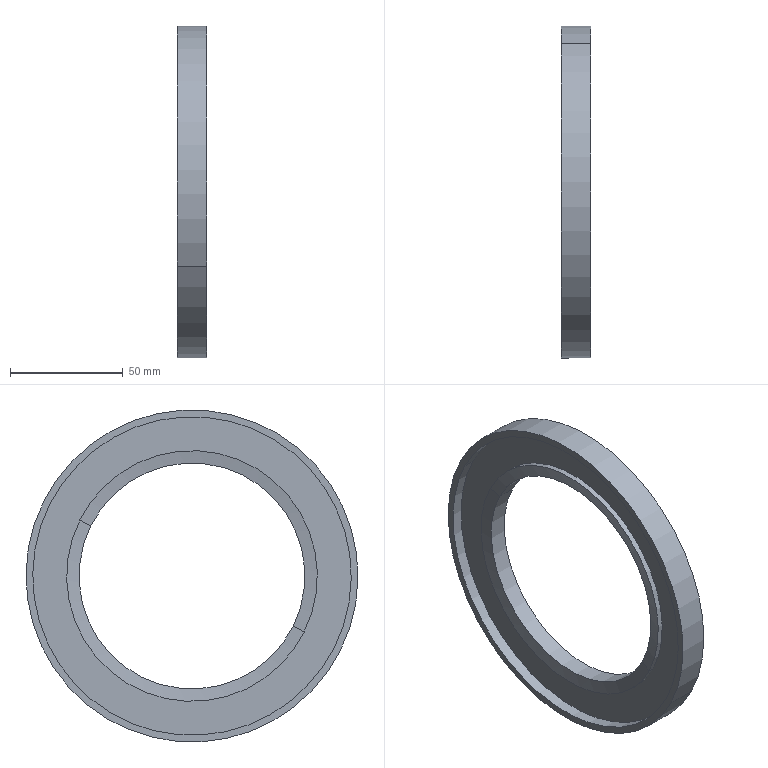Component | SolidWorks | SpringSeat-1 | 1 solid | 16 faces | box 13 x 147 x 147 mm | volume 74131 mm3 | cylinder 10 | plane 4 | cone 2 | commonest cylinder face diameters 141 x2 111 x2 100 x2 134 x2 147 x2
build123d program:
from build123d import *


with BuildPart() as part:
    # Sketch1 → Revolve1 (revolve)
    with BuildSketch(Plane.XY, mode=Mode.PRIVATE) as revolve1_sk:
        Polygon((0, 73.5), (13, 73.5), (13, 67), (11.5, 67), (11.5, 50), (3.371, 50), (2.5, 55.5), (5, 55.5), (5, 70.5), (0, 70.5), align=None)
    revolve(revolve1_sk.sketch.rotate(Axis((0, 0, 0), (1, 0, 0)), 90), axis=Axis((0, 0, 0), (1, 0, 0)))


solid = part.part

# Placed as in the assembly
solid = solid.moved(Location((-149.5, 0, 0), (0, 0, 0)))
STEP:
#1=COLOUR_RGB('',0.7922,0.8196,0.9333);
#2=FILL_AREA_STYLE_COLOUR('',#1);
#3=FILL_AREA_STYLE('',(#2));
#4=SURFACE_STYLE_FILL_AREA(#3);
#5=SURFACE_SIDE_STYLE('',(#4));
#6=SURFACE_STYLE_USAGE(.BOTH.,#5);
#7=PRESENTATION_STYLE_ASSIGNMENT((#6));
#8=CARTESIAN_POINT('',(-5.689,-2.483,-1.24));
#9=VERTEX_POINT('',#8);
#10=CARTESIAN_POINT('',(-5.689,2.483,1.24));
#11=VERTEX_POINT('',#10);
#12=CARTESIAN_POINT('',(-5.689,-0.,0.));
#13=DIRECTION('',(-1.,-0.,0.));
#14=DIRECTION('',(-0.,0.8946,0.4468));
#15=AXIS2_PLACEMENT_3D('',#12,#13,#14);
#16=CIRCLE('',#15,2.776);
#17=EDGE_CURVE('',#9,#11,#16,.T.);
#18=ORIENTED_EDGE('',*,*,#17,.F.);
#19=CARTESIAN_POINT('',(-5.886,-2.483,-1.24));
#20=VERTEX_POINT('',#19);
#21=CARTESIAN_POINT('',(-5.886,-2.483,-1.24));
#22=DIRECTION('',(-1.,-0.,0.));
#23=VECTOR('',#22,39.37);
#24=LINE('',#21,#23);
#25=EDGE_CURVE('',#9,#20,#24,.T.);
#26=ORIENTED_EDGE('',*,*,#25,.T.);
#27=CARTESIAN_POINT('',(-5.886,2.483,1.24));
#28=VERTEX_POINT('',#27);
#29=CARTESIAN_POINT('',(-5.886,-0.,0.));
#30=DIRECTION('',(-1.,-0.,0.));
#31=DIRECTION('',(-0.,0.8946,0.4468));
#32=AXIS2_PLACEMENT_3D('',#29,#30,#31);
#33=CIRCLE('',#32,2.776);
#34=EDGE_CURVE('',#20,#28,#33,.T.);
#35=ORIENTED_EDGE('',*,*,#34,.T.);
#36=CARTESIAN_POINT('',(-5.886,2.483,1.24));
#37=DIRECTION('',(-1.,-0.,0.));
#38=VECTOR('',#37,39.37);
#39=LINE('',#36,#38);
#40=EDGE_CURVE('',#11,#28,#39,.T.);
#41=ORIENTED_EDGE('',*,*,#40,.F.);
#42=EDGE_LOOP('',(#18,#26,#35,#41));
#43=FACE_OUTER_BOUND('',#42,.T.);
#44=CARTESIAN_POINT('',(-5.886,-0.,0.));
#45=DIRECTION('',(-1.,-0.,0.));
#46=DIRECTION('',(-0.,0.8946,0.4468));
#47=AXIS2_PLACEMENT_3D('',#44,#45,#46);
#48=CYLINDRICAL_SURFACE('',#47,2.776);
#49=ADVANCED_FACE('',(#43),#48,.F.);
#50=CARTESIAN_POINT('',(-5.689,1.955,0.9764));
#51=VERTEX_POINT('',#50);
#52=CARTESIAN_POINT('',(-5.689,-1.955,-0.9764));
#53=VERTEX_POINT('',#52);
#54=CARTESIAN_POINT('',(-5.689,-0.,0.));
#55=DIRECTION('',(-1.,-0.,0.));
#56=DIRECTION('',(-0.,0.8946,0.4468));
#57=AXIS2_PLACEMENT_3D('',#54,#55,#56);
#58=CIRCLE('',#57,2.185);
#59=EDGE_CURVE('',#51,#53,#58,.T.);
#60=ORIENTED_EDGE('',*,*,#59,.T.);
#61=CARTESIAN_POINT('',(-5.787,-1.955,-0.9764));
#62=VERTEX_POINT('',#61);
#63=CARTESIAN_POINT('',(-5.886,-1.955,-0.9764));
#64=DIRECTION('',(-1.,-0.,0.));
#65=VECTOR('',#64,39.37);
#66=LINE('',#63,#65);
#67=EDGE_CURVE('',#53,#62,#66,.T.);
#68=ORIENTED_EDGE('',*,*,#67,.T.);
#69=CARTESIAN_POINT('',(-5.787,1.955,0.9764));
#70=VERTEX_POINT('',#69);
#71=CARTESIAN_POINT('',(-5.787,-0.,0.));
#72=DIRECTION('',(-1.,-0.,0.));
#73=DIRECTION('',(-0.,0.8946,0.4468));
#74=AXIS2_PLACEMENT_3D('',#71,#72,#73);
#75=CIRCLE('',#74,2.185);
#76=EDGE_CURVE('',#70,#62,#75,.T.);
#77=ORIENTED_EDGE('',*,*,#76,.F.);
#78=CARTESIAN_POINT('',(-5.886,1.955,0.9764));
#79=DIRECTION('',(-1.,-0.,0.));
#80=VECTOR('',#79,39.37);
#81=LINE('',#78,#80);
#82=EDGE_CURVE('',#51,#70,#81,.T.);
#83=ORIENTED_EDGE('',*,*,#82,.F.);
#84=EDGE_LOOP('',(#60,#68,#77,#83));
#85=FACE_OUTER_BOUND('',#84,.T.);
#86=CARTESIAN_POINT('',(-5.886,-0.,0.));
#87=DIRECTION('',(-1.,-0.,0.));
#88=DIRECTION('',(-0.,0.8946,0.4468));
#89=AXIS2_PLACEMENT_3D('',#86,#87,#88);
#90=CYLINDRICAL_SURFACE('',#89,2.185);
#91=ADVANCED_FACE('',(#85),#90,.T.);
#92=CARTESIAN_POINT('',(-5.753,-1.761,-0.8796));
#93=VERTEX_POINT('',#92);
#94=CARTESIAN_POINT('',(-5.753,1.761,0.8796));
#95=VERTEX_POINT('',#94);
#96=CARTESIAN_POINT('',(-5.753,-0.,0.));
#97=DIRECTION('',(-1.,-0.,0.));
#98=DIRECTION('',(-0.,0.8946,0.4468));
#99=AXIS2_PLACEMENT_3D('',#96,#97,#98);
#100=CIRCLE('',#99,1.969);
#101=EDGE_CURVE('',#93,#95,#100,.T.);
#102=ORIENTED_EDGE('',*,*,#101,.F.);
#103=CARTESIAN_POINT('',(-5.787,-1.955,-0.9764));
#104=DIRECTION('',(-0.1564,-0.8836,-0.4413));
#105=VECTOR('',#104,39.37);
#106=LINE('',#103,#105);
#107=EDGE_CURVE('',#93,#62,#106,.T.);
#108=ORIENTED_EDGE('',*,*,#107,.T.);
#109=CARTESIAN_POINT('',(-5.787,-0.,0.));
#110=DIRECTION('',(-1.,-0.,0.));
#111=DIRECTION('',(-0.,0.8946,0.4468));
#112=AXIS2_PLACEMENT_3D('',#109,#110,#111);
#113=CIRCLE('',#112,2.185);
#114=EDGE_CURVE('',#62,#70,#113,.T.);
#115=ORIENTED_EDGE('',*,*,#114,.T.);
#116=CARTESIAN_POINT('',(-5.787,1.955,0.9764));
#117=DIRECTION('',(-0.1564,0.8836,0.4413));
#118=VECTOR('',#117,39.37);
#119=LINE('',#116,#118);
#120=EDGE_CURVE('',#95,#70,#119,.T.);
#121=ORIENTED_EDGE('',*,*,#120,.F.);
#122=EDGE_LOOP('',(#102,#108,#115,#121));
#123=FACE_OUTER_BOUND('',#122,.T.);
#124=CARTESIAN_POINT('',(-5.787,-0.,0.));
#125=DIRECTION('',(-1.,-0.,0.));
#126=DIRECTION('',(-0.,0.8946,0.4468));
#127=AXIS2_PLACEMENT_3D('',#124,#125,#126);
#128=CONICAL_SURFACE('',#127,2.185,1.414);
#129=ADVANCED_FACE('',(#123),#128,.F.);
#130=CARTESIAN_POINT('',(-5.433,-1.761,-0.8796));
#131=VERTEX_POINT('',#130);
#132=CARTESIAN_POINT('',(-5.433,1.761,0.8796));
#133=VERTEX_POINT('',#132);
#134=CARTESIAN_POINT('',(-5.433,-0.,0.));
#135=DIRECTION('',(-1.,-0.,0.));
#136=DIRECTION('',(-0.,0.8946,0.4468));
#137=AXIS2_PLACEMENT_3D('',#134,#135,#136);
#138=CIRCLE('',#137,1.969);
#139=EDGE_CURVE('',#131,#133,#138,.T.);
#140=ORIENTED_EDGE('',*,*,#139,.F.);
#141=CARTESIAN_POINT('',(-5.886,-1.761,-0.8796));
#142=DIRECTION('',(-1.,-0.,0.));
#143=VECTOR('',#142,39.37);
#144=LINE('',#141,#143);
#145=EDGE_CURVE('',#131,#93,#144,.T.);
#146=ORIENTED_EDGE('',*,*,#145,.T.);
#147=ORIENTED_EDGE('',*,*,#101,.T.);
#148=CARTESIAN_POINT('',(-5.886,1.761,0.8796));
#149=DIRECTION('',(-1.,-0.,0.));
#150=VECTOR('',#149,39.37);
#151=LINE('',#148,#150);
#152=EDGE_CURVE('',#133,#95,#151,.T.);
#153=ORIENTED_EDGE('',*,*,#152,.F.);
#154=EDGE_LOOP('',(#140,#146,#147,#153));
#155=FACE_OUTER_BOUND('',#154,.T.);
#156=CARTESIAN_POINT('',(-5.886,-0.,0.));
#157=DIRECTION('',(-1.,-0.,0.));
#158=DIRECTION('',(-0.,0.8946,0.4468));
#159=AXIS2_PLACEMENT_3D('',#156,#157,#158);
#160=CYLINDRICAL_SURFACE('',#159,1.969);
#161=ADVANCED_FACE('',(#155),#160,.F.);
#162=CARTESIAN_POINT('',(-5.374,-2.36,-1.179));
#163=VERTEX_POINT('',#162);
#164=CARTESIAN_POINT('',(-5.374,2.36,1.179));
#165=VERTEX_POINT('',#164);
#166=CARTESIAN_POINT('',(-5.374,-0.,0.));
#167=DIRECTION('',(-1.,-0.,0.));
#168=DIRECTION('',(-0.,0.8946,0.4468));
#169=AXIS2_PLACEMENT_3D('',#166,#167,#168);
#170=CIRCLE('',#169,2.638);
#171=EDGE_CURVE('',#163,#165,#170,.T.);
#172=ORIENTED_EDGE('',*,*,#171,.F.);
#173=CARTESIAN_POINT('',(-5.433,-2.36,-1.179));
#174=VERTEX_POINT('',#173);
#175=CARTESIAN_POINT('',(-5.886,-2.36,-1.179));
#176=DIRECTION('',(-1.,-0.,0.));
#177=VECTOR('',#176,39.37);
#178=LINE('',#175,#177);
#179=EDGE_CURVE('',#163,#174,#178,.T.);
#180=ORIENTED_EDGE('',*,*,#179,.T.);
#181=CARTESIAN_POINT('',(-5.433,2.36,1.179));
#182=VERTEX_POINT('',#181);
#183=CARTESIAN_POINT('',(-5.433,-0.,0.));
#184=DIRECTION('',(-1.,-0.,0.));
#185=DIRECTION('',(-0.,0.8946,0.4468));
#186=AXIS2_PLACEMENT_3D('',#183,#184,#185);
#187=CIRCLE('',#186,2.638);
#188=EDGE_CURVE('',#174,#182,#187,.T.);
#189=ORIENTED_EDGE('',*,*,#188,.T.);
#190=CARTESIAN_POINT('',(-5.886,2.36,1.179));
#191=DIRECTION('',(-1.,-0.,0.));
#192=VECTOR('',#191,39.37);
#193=LINE('',#190,#192);
#194=EDGE_CURVE('',#165,#182,#193,.T.);
#195=ORIENTED_EDGE('',*,*,#194,.F.);
#196=EDGE_LOOP('',(#172,#180,#189,#195));
#197=FACE_OUTER_BOUND('',#196,.T.);
#198=CARTESIAN_POINT('',(-5.886,-0.,0.));
#199=DIRECTION('',(-1.,-0.,0.));
#200=DIRECTION('',(-0.,0.8946,0.4468));
#201=AXIS2_PLACEMENT_3D('',#198,#199,#200);
#202=CYLINDRICAL_SURFACE('',#201,2.638);
#203=ADVANCED_FACE('',(#197),#202,.F.);
#204=CARTESIAN_POINT('',(-5.374,2.589,1.293));
#205=VERTEX_POINT('',#204);
#206=CARTESIAN_POINT('',(-5.374,-2.589,-1.293));
#207=VERTEX_POINT('',#206);
#208=CARTESIAN_POINT('',(-5.374,-0.,0.));
#209=DIRECTION('',(-1.,-0.,0.));
#210=DIRECTION('',(-0.,0.8946,0.4468));
#211=AXIS2_PLACEMENT_3D('',#208,#209,#210);
#212=CIRCLE('',#211,2.894);
#213=EDGE_CURVE('',#205,#207,#212,.T.);
#214=ORIENTED_EDGE('',*,*,#213,.T.);
#215=CARTESIAN_POINT('',(-5.886,-2.589,-1.293));
#216=VERTEX_POINT('',#215);
#217=CARTESIAN_POINT('',(-5.886,-2.589,-1.293));
#218=DIRECTION('',(-1.,-0.,0.));
#219=VECTOR('',#218,39.37);
#220=LINE('',#217,#219);
#221=EDGE_CURVE('',#207,#216,#220,.T.);
#222=ORIENTED_EDGE('',*,*,#221,.T.);
#223=CARTESIAN_POINT('',(-5.886,2.589,1.293));
#224=VERTEX_POINT('',#223);
#225=CARTESIAN_POINT('',(-5.886,-0.,0.));
#226=DIRECTION('',(-1.,-0.,0.));
#227=DIRECTION('',(-0.,0.8946,0.4468));
#228=AXIS2_PLACEMENT_3D('',#225,#226,#227);
#229=CIRCLE('',#228,2.894);
#230=EDGE_CURVE('',#224,#216,#229,.T.);
#231=ORIENTED_EDGE('',*,*,#230,.F.);
#232=CARTESIAN_POINT('',(-5.886,2.589,1.293));
#233=DIRECTION('',(-1.,-0.,0.));
#234=VECTOR('',#233,39.37);
#235=LINE('',#232,#234);
#236=EDGE_CURVE('',#205,#224,#235,.T.);
#237=ORIENTED_EDGE('',*,*,#236,.F.);
#238=EDGE_LOOP('',(#214,#222,#231,#237));
#239=FACE_OUTER_BOUND('',#238,.T.);
#240=CARTESIAN_POINT('',(-5.886,-0.,0.));
#241=DIRECTION('',(-1.,-0.,0.));
#242=DIRECTION('',(-0.,0.8946,0.4468));
#243=AXIS2_PLACEMENT_3D('',#240,#241,#242);
#244=CYLINDRICAL_SURFACE('',#243,2.894);
#245=ADVANCED_FACE('',(#239),#244,.T.);
#246=CARTESIAN_POINT('',(-5.886,-0.,0.));
#247=DIRECTION('',(-1.,-0.,0.));
#248=DIRECTION('',(-0.,0.8946,0.4468));
#249=AXIS2_PLACEMENT_3D('',#246,#247,#248);
#250=CIRCLE('',#249,2.776);
#251=EDGE_CURVE('',#28,#20,#250,.T.);
#252=ORIENTED_EDGE('',*,*,#251,.F.);
#253=ORIENTED_EDGE('',*,*,#34,.F.);
#254=EDGE_LOOP('',(#252,#253));
#255=FACE_BOUND('',#254,.T.);
#256=ORIENTED_EDGE('',*,*,#230,.T.);
#257=CARTESIAN_POINT('',(-5.886,-0.,0.));
#258=DIRECTION('',(-1.,-0.,0.));
#259=DIRECTION('',(-0.,0.8946,0.4468));
#260=AXIS2_PLACEMENT_3D('',#257,#258,#259);
#261=CIRCLE('',#260,2.894);
#262=EDGE_CURVE('',#216,#224,#261,.T.);
#263=ORIENTED_EDGE('',*,*,#262,.T.);
#264=EDGE_LOOP('',(#256,#263));
#265=FACE_OUTER_BOUND('',#264,.T.);
#266=CARTESIAN_POINT('',(-5.886,1.24,-2.483));
#267=DIRECTION('',(1.,0.,-0.));
#268=DIRECTION('',(0.,-0.8946,-0.4468));
#269=AXIS2_PLACEMENT_3D('',#266,#267,#268);
#270=PLANE('',#269);
#271=ADVANCED_FACE('',(#255,#265),#270,.F.);
#272=ORIENTED_EDGE('',*,*,#221,.F.);
#273=CARTESIAN_POINT('',(-5.374,-0.,0.));
#274=DIRECTION('',(-1.,-0.,0.));
#275=DIRECTION('',(-0.,0.8946,0.4468));
#276=AXIS2_PLACEMENT_3D('',#273,#274,#275);
#277=CIRCLE('',#276,2.894);
#278=EDGE_CURVE('',#207,#205,#277,.T.);
#279=ORIENTED_EDGE('',*,*,#278,.T.);
#280=ORIENTED_EDGE('',*,*,#236,.T.);
#281=ORIENTED_EDGE('',*,*,#262,.F.);
#282=EDGE_LOOP('',(#272,#279,#280,#281));
#283=FACE_OUTER_BOUND('',#282,.T.);
#284=CARTESIAN_POINT('',(-5.886,-0.,0.));
#285=DIRECTION('',(-1.,-0.,0.));
#286=DIRECTION('',(-0.,0.8946,0.4468));
#287=AXIS2_PLACEMENT_3D('',#284,#285,#286);
#288=CYLINDRICAL_SURFACE('',#287,2.894);
#289=ADVANCED_FACE('',(#283),#288,.T.);
#290=ORIENTED_EDGE('',*,*,#213,.F.);
#291=ORIENTED_EDGE('',*,*,#278,.F.);
#292=EDGE_LOOP('',(#290,#291));
#293=FACE_OUTER_BOUND('',#292,.T.);
#294=CARTESIAN_POINT('',(-5.374,-0.,0.));
#295=DIRECTION('',(-1.,-0.,0.));
#296=DIRECTION('',(-0.,0.8946,0.4468));
#297=AXIS2_PLACEMENT_3D('',#294,#295,#296);
#298=CIRCLE('',#297,2.638);
#299=EDGE_CURVE('',#165,#163,#298,.T.);
#300=ORIENTED_EDGE('',*,*,#299,.T.);
#301=ORIENTED_EDGE('',*,*,#171,.T.);
#302=EDGE_LOOP('',(#300,#301));
#303=FACE_BOUND('',#302,.T.);
#304=CARTESIAN_POINT('',(-5.374,1.293,-2.589));
#305=DIRECTION('',(-1.,-0.,0.));
#306=DIRECTION('',(-0.,0.8946,0.4468));
#307=AXIS2_PLACEMENT_3D('',#304,#305,#306);
#308=PLANE('',#307);
#309=ADVANCED_FACE('',(#293,#303),#308,.F.);
#310=ORIENTED_EDGE('',*,*,#179,.F.);
#311=ORIENTED_EDGE('',*,*,#299,.F.);
#312=ORIENTED_EDGE('',*,*,#194,.T.);
#313=CARTESIAN_POINT('',(-5.433,-0.,0.));
#314=DIRECTION('',(-1.,-0.,0.));
#315=DIRECTION('',(-0.,0.8946,0.4468));
#316=AXIS2_PLACEMENT_3D('',#313,#314,#315);
#317=CIRCLE('',#316,2.638);
#318=EDGE_CURVE('',#182,#174,#317,.T.);
#319=ORIENTED_EDGE('',*,*,#318,.T.);
#320=EDGE_LOOP('',(#310,#311,#312,#319));
#321=FACE_OUTER_BOUND('',#320,.T.);
#322=CARTESIAN_POINT('',(-5.886,-0.,0.));
#323=DIRECTION('',(-1.,-0.,0.));
#324=DIRECTION('',(-0.,0.8946,0.4468));
#325=AXIS2_PLACEMENT_3D('',#322,#323,#324);
#326=CYLINDRICAL_SURFACE('',#325,2.638);
#327=ADVANCED_FACE('',(#321),#326,.F.);
#328=ORIENTED_EDGE('',*,*,#318,.F.);
#329=ORIENTED_EDGE('',*,*,#188,.F.);
#330=EDGE_LOOP('',(#328,#329));
#331=FACE_OUTER_BOUND('',#330,.T.);
#332=CARTESIAN_POINT('',(-5.433,-0.,0.));
#333=DIRECTION('',(-1.,-0.,0.));
#334=DIRECTION('',(-0.,0.8946,0.4468));
#335=AXIS2_PLACEMENT_3D('',#332,#333,#334);
#336=CIRCLE('',#335,1.969);
#337=EDGE_CURVE('',#133,#131,#336,.T.);
#338=ORIENTED_EDGE('',*,*,#337,.T.);
#339=ORIENTED_EDGE('',*,*,#139,.T.);
#340=EDGE_LOOP('',(#338,#339));
#341=FACE_BOUND('',#340,.T.);
#342=CARTESIAN_POINT('',(-5.433,1.179,-2.36));
#343=DIRECTION('',(-1.,-0.,0.));
#344=DIRECTION('',(-0.,0.8946,0.4468));
#345=AXIS2_PLACEMENT_3D('',#342,#343,#344);
#346=PLANE('',#345);
#347=ADVANCED_FACE('',(#331,#341),#346,.F.);
#348=ORIENTED_EDGE('',*,*,#145,.F.);
#349=ORIENTED_EDGE('',*,*,#337,.F.);
#350=ORIENTED_EDGE('',*,*,#152,.T.);
#351=CARTESIAN_POINT('',(-5.753,-0.,0.));
#352=DIRECTION('',(-1.,-0.,0.));
#353=DIRECTION('',(-0.,0.8946,0.4468));
#354=AXIS2_PLACEMENT_3D('',#351,#352,#353);
#355=CIRCLE('',#354,1.969);
#356=EDGE_CURVE('',#95,#93,#355,.T.);
#357=ORIENTED_EDGE('',*,*,#356,.T.);
#358=EDGE_LOOP('',(#348,#349,#350,#357));
#359=FACE_OUTER_BOUND('',#358,.T.);
#360=CARTESIAN_POINT('',(-5.886,-0.,0.));
#361=DIRECTION('',(-1.,-0.,0.));
#362=DIRECTION('',(-0.,0.8946,0.4468));
#363=AXIS2_PLACEMENT_3D('',#360,#361,#362);
#364=CYLINDRICAL_SURFACE('',#363,1.969);
#365=ADVANCED_FACE('',(#359),#364,.F.);
#366=ORIENTED_EDGE('',*,*,#107,.F.);
#367=ORIENTED_EDGE('',*,*,#356,.F.);
#368=ORIENTED_EDGE('',*,*,#120,.T.);
#369=ORIENTED_EDGE('',*,*,#76,.T.);
#370=EDGE_LOOP('',(#366,#367,#368,#369));
#371=FACE_OUTER_BOUND('',#370,.T.);
#372=CARTESIAN_POINT('',(-5.787,-0.,0.));
#373=DIRECTION('',(-1.,-0.,0.));
#374=DIRECTION('',(-0.,0.8946,0.4468));
#375=AXIS2_PLACEMENT_3D('',#372,#373,#374);
#376=CONICAL_SURFACE('',#375,2.185,1.414);
#377=ADVANCED_FACE('',(#371),#376,.F.);
#378=ORIENTED_EDGE('',*,*,#67,.F.);
#379=CARTESIAN_POINT('',(-5.689,-0.,0.));
#380=DIRECTION('',(-1.,-0.,0.));
#381=DIRECTION('',(-0.,0.8946,0.4468));
#382=AXIS2_PLACEMENT_3D('',#379,#380,#381);
#383=CIRCLE('',#382,2.185);
#384=EDGE_CURVE('',#53,#51,#383,.T.);
#385=ORIENTED_EDGE('',*,*,#384,.T.);
#386=ORIENTED_EDGE('',*,*,#82,.T.);
#387=ORIENTED_EDGE('',*,*,#114,.F.);
#388=EDGE_LOOP('',(#378,#385,#386,#387));
#389=FACE_OUTER_BOUND('',#388,.T.);
#390=CARTESIAN_POINT('',(-5.886,-0.,0.));
#391=DIRECTION('',(-1.,-0.,0.));
#392=DIRECTION('',(-0.,0.8946,0.4468));
#393=AXIS2_PLACEMENT_3D('',#390,#391,#392);
#394=CYLINDRICAL_SURFACE('',#393,2.185);
#395=ADVANCED_FACE('',(#389),#394,.T.);
#396=ORIENTED_EDGE('',*,*,#59,.F.);
#397=ORIENTED_EDGE('',*,*,#384,.F.);
#398=EDGE_LOOP('',(#396,#397));
#399=FACE_BOUND('',#398,.T.);
#400=CARTESIAN_POINT('',(-5.689,-0.,0.));
#401=DIRECTION('',(-1.,-0.,0.));
#402=DIRECTION('',(-0.,0.8946,0.4468));
#403=AXIS2_PLACEMENT_3D('',#400,#401,#402);
#404=CIRCLE('',#403,2.776);
#405=EDGE_CURVE('',#11,#9,#404,.T.);
#406=ORIENTED_EDGE('',*,*,#405,.T.);
#407=ORIENTED_EDGE('',*,*,#17,.T.);
#408=EDGE_LOOP('',(#406,#407));
#409=FACE_OUTER_BOUND('',#408,.T.);
#410=CARTESIAN_POINT('',(-5.689,0.9764,-1.955));
#411=DIRECTION('',(1.,0.,-0.));
#412=DIRECTION('',(0.,-0.8946,-0.4468));
#413=AXIS2_PLACEMENT_3D('',#410,#411,#412);
#414=PLANE('',#413);
#415=ADVANCED_FACE('',(#399,#409),#414,.F.);
#416=ORIENTED_EDGE('',*,*,#25,.F.);
#417=ORIENTED_EDGE('',*,*,#405,.F.);
#418=ORIENTED_EDGE('',*,*,#40,.T.);
#419=ORIENTED_EDGE('',*,*,#251,.T.);
#420=EDGE_LOOP('',(#416,#417,#418,#419));
#421=FACE_OUTER_BOUND('',#420,.T.);
#422=CARTESIAN_POINT('',(-5.886,-0.,0.));
#423=DIRECTION('',(-1.,-0.,0.));
#424=DIRECTION('',(-0.,0.8946,0.4468));
#425=AXIS2_PLACEMENT_3D('',#422,#423,#424);
#426=CYLINDRICAL_SURFACE('',#425,2.776);
#427=ADVANCED_FACE('',(#421),#426,.F.);
#428=CLOSED_SHELL('',(#49,#91,#129,#161,#203,#245,#271,#289,#309,#327,#347,#365,#377,#395,#415,#427));
#429=MANIFOLD_SOLID_BREP('',#428);
#430=STYLED_ITEM('',(#7),#429);
#431=PRESENTATION_LAYER_ASSIGNMENT('','',(#430));
#432=CARTESIAN_POINT('',(0.,0.,0.));
#433=DIRECTION('',(0.,0.,1.));
#434=DIRECTION('',(1.,0.,0.));
#435=AXIS2_PLACEMENT_3D('',#432,#433,#434);
#436=(LENGTH_UNIT()NAMED_UNIT(*)SI_UNIT($,.METRE.));
#437=LENGTH_MEASURE_WITH_UNIT(LENGTH_MEASURE(0.0254),#436);
#438=DIMENSIONAL_EXPONENTS(1.,0.,0.,0.,0.,0.,0.);
#439=(CONVERSION_BASED_UNIT('',#437)LENGTH_UNIT()NAMED_UNIT(#438));
#440=UNCERTAINTY_MEASURE_WITH_UNIT(LENGTH_MEASURE(0.00001),#439,'','');
#441=(NAMED_UNIT(*)PLANE_ANGLE_UNIT()SI_UNIT($,.RADIAN.));
#442=(NAMED_UNIT(*)SI_UNIT($,.STERADIAN.)SOLID_ANGLE_UNIT());
#443=(GEOMETRIC_REPRESENTATION_CONTEXT(3)GLOBAL_UNCERTAINTY_ASSIGNED_CONTEXT((#440))GLOBAL_UNIT_ASSIGNED_CONTEXT((#439,#441,#442))REPRESENTATION_CONTEXT('',''));
#444=ADVANCED_BREP_SHAPE_REPRESENTATION('',(#429,#435),#443);
#445=(LENGTH_UNIT()NAMED_UNIT(*)SI_UNIT($,.METRE.));
#446=LENGTH_MEASURE_WITH_UNIT(LENGTH_MEASURE(0.0254),#445);
#447=DIMENSIONAL_EXPONENTS(1.,0.,0.,0.,0.,0.,0.);
#448=(CONVERSION_BASED_UNIT('',#446)LENGTH_UNIT()NAMED_UNIT(#447));
#449=UNCERTAINTY_MEASURE_WITH_UNIT(LENGTH_MEASURE(0.00001),#448,'','');
#450=(NAMED_UNIT(*)PLANE_ANGLE_UNIT()SI_UNIT($,.RADIAN.));
#451=(NAMED_UNIT(*)SI_UNIT($,.STERADIAN.)SOLID_ANGLE_UNIT());
#452=(GEOMETRIC_REPRESENTATION_CONTEXT(3)GLOBAL_UNCERTAINTY_ASSIGNED_CONTEXT((#449))GLOBAL_UNIT_ASSIGNED_CONTEXT((#448,#450,#451))REPRESENTATION_CONTEXT('',''));
#453=MECHANICAL_DESIGN_GEOMETRIC_PRESENTATION_REPRESENTATION('',(#430),#452);